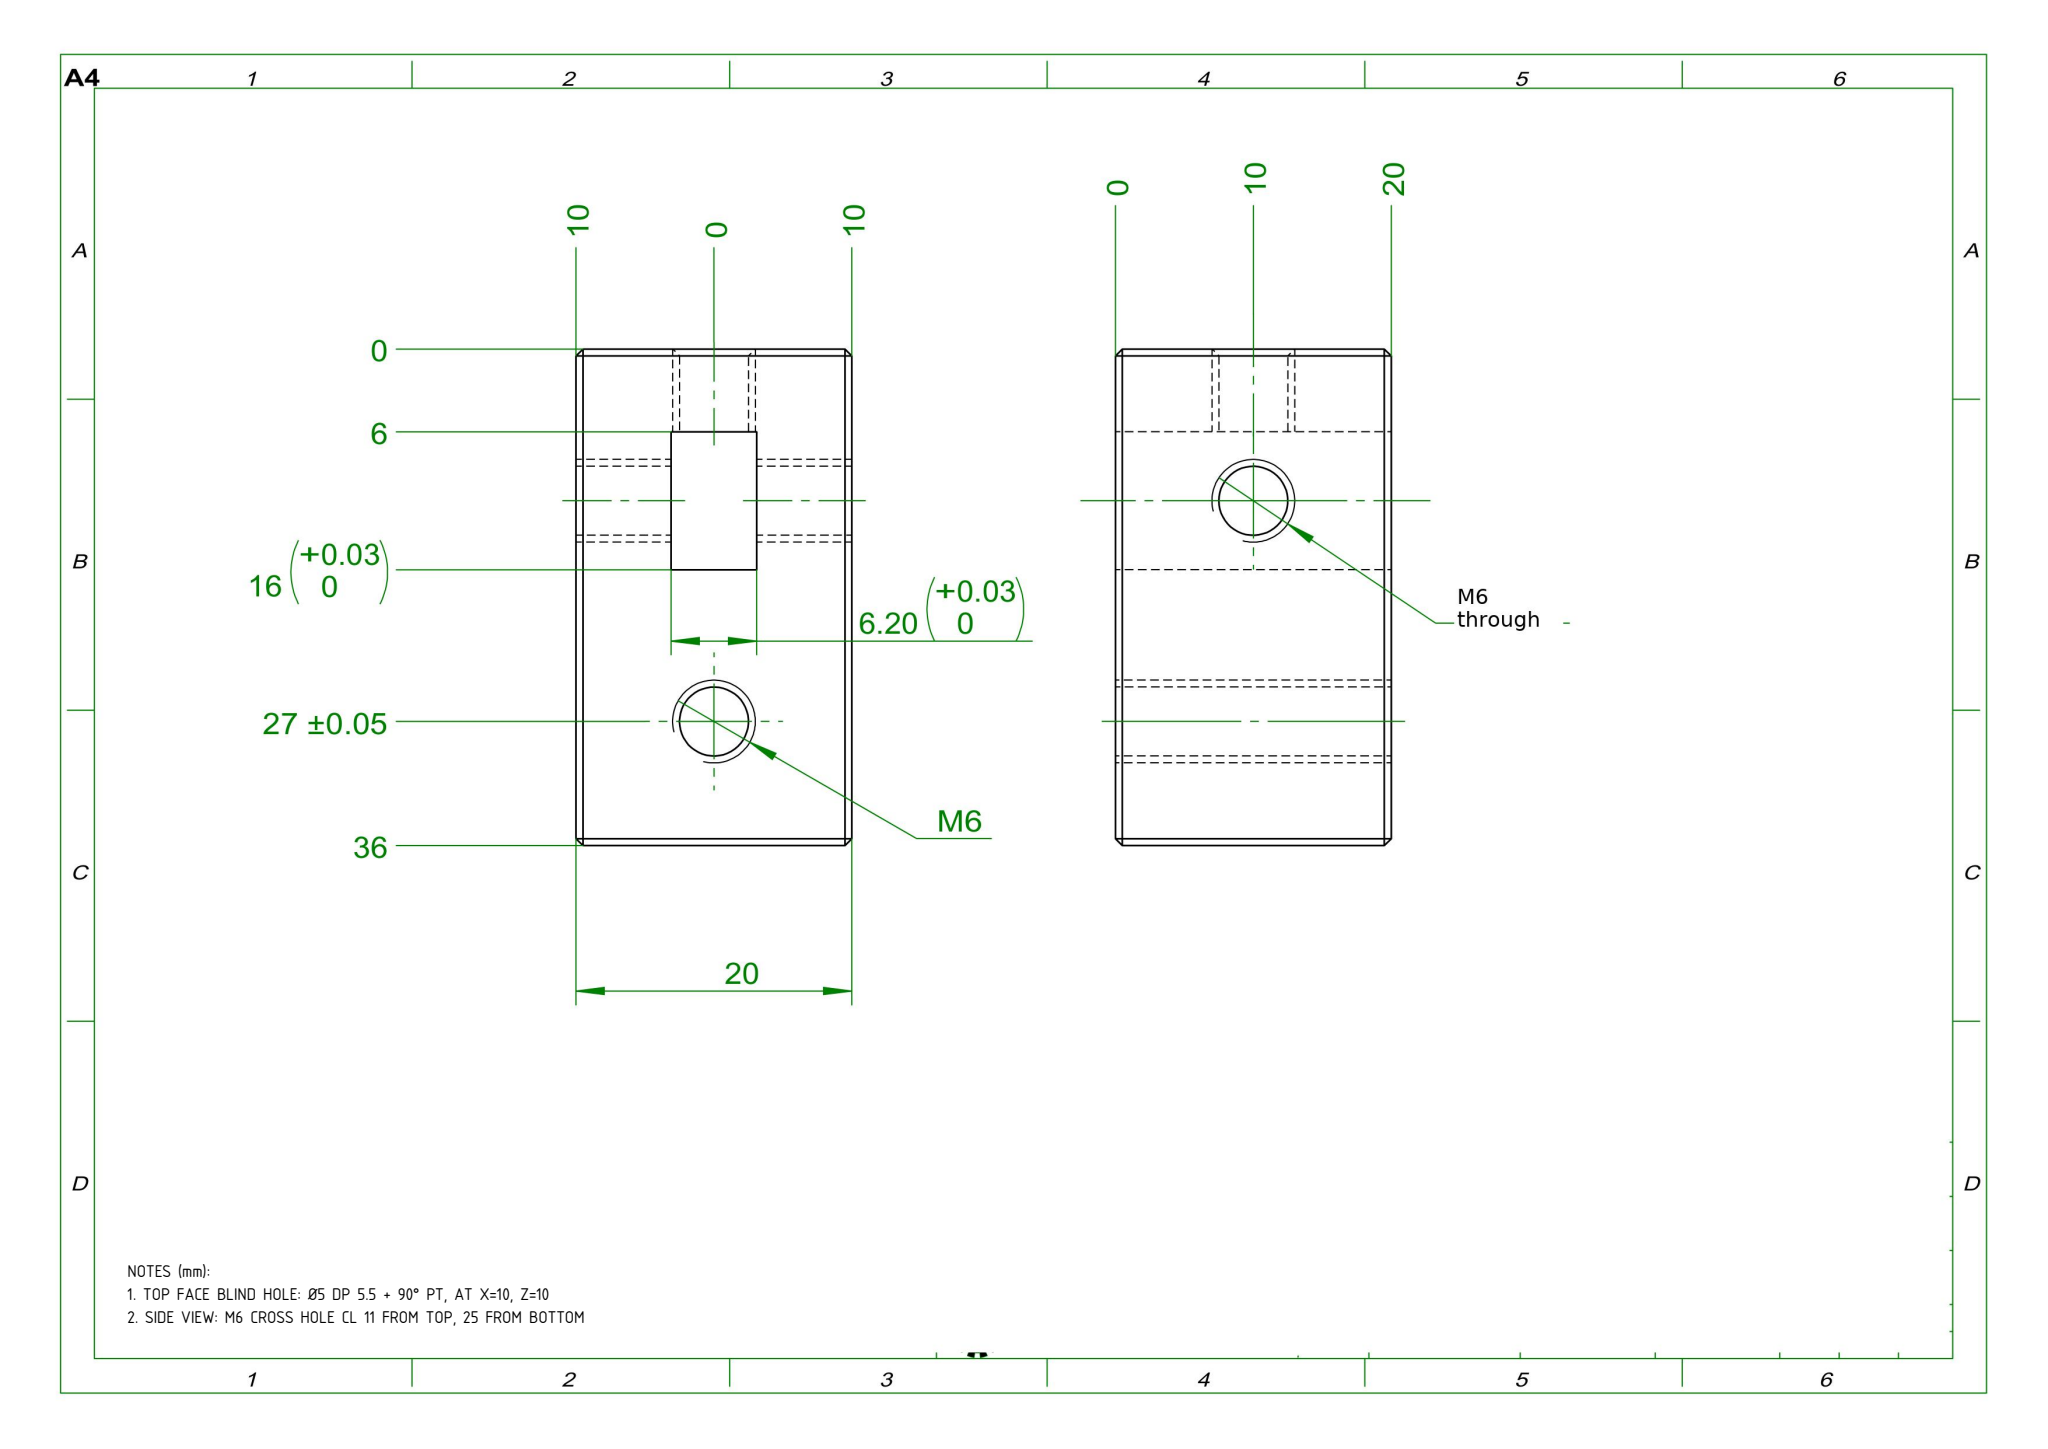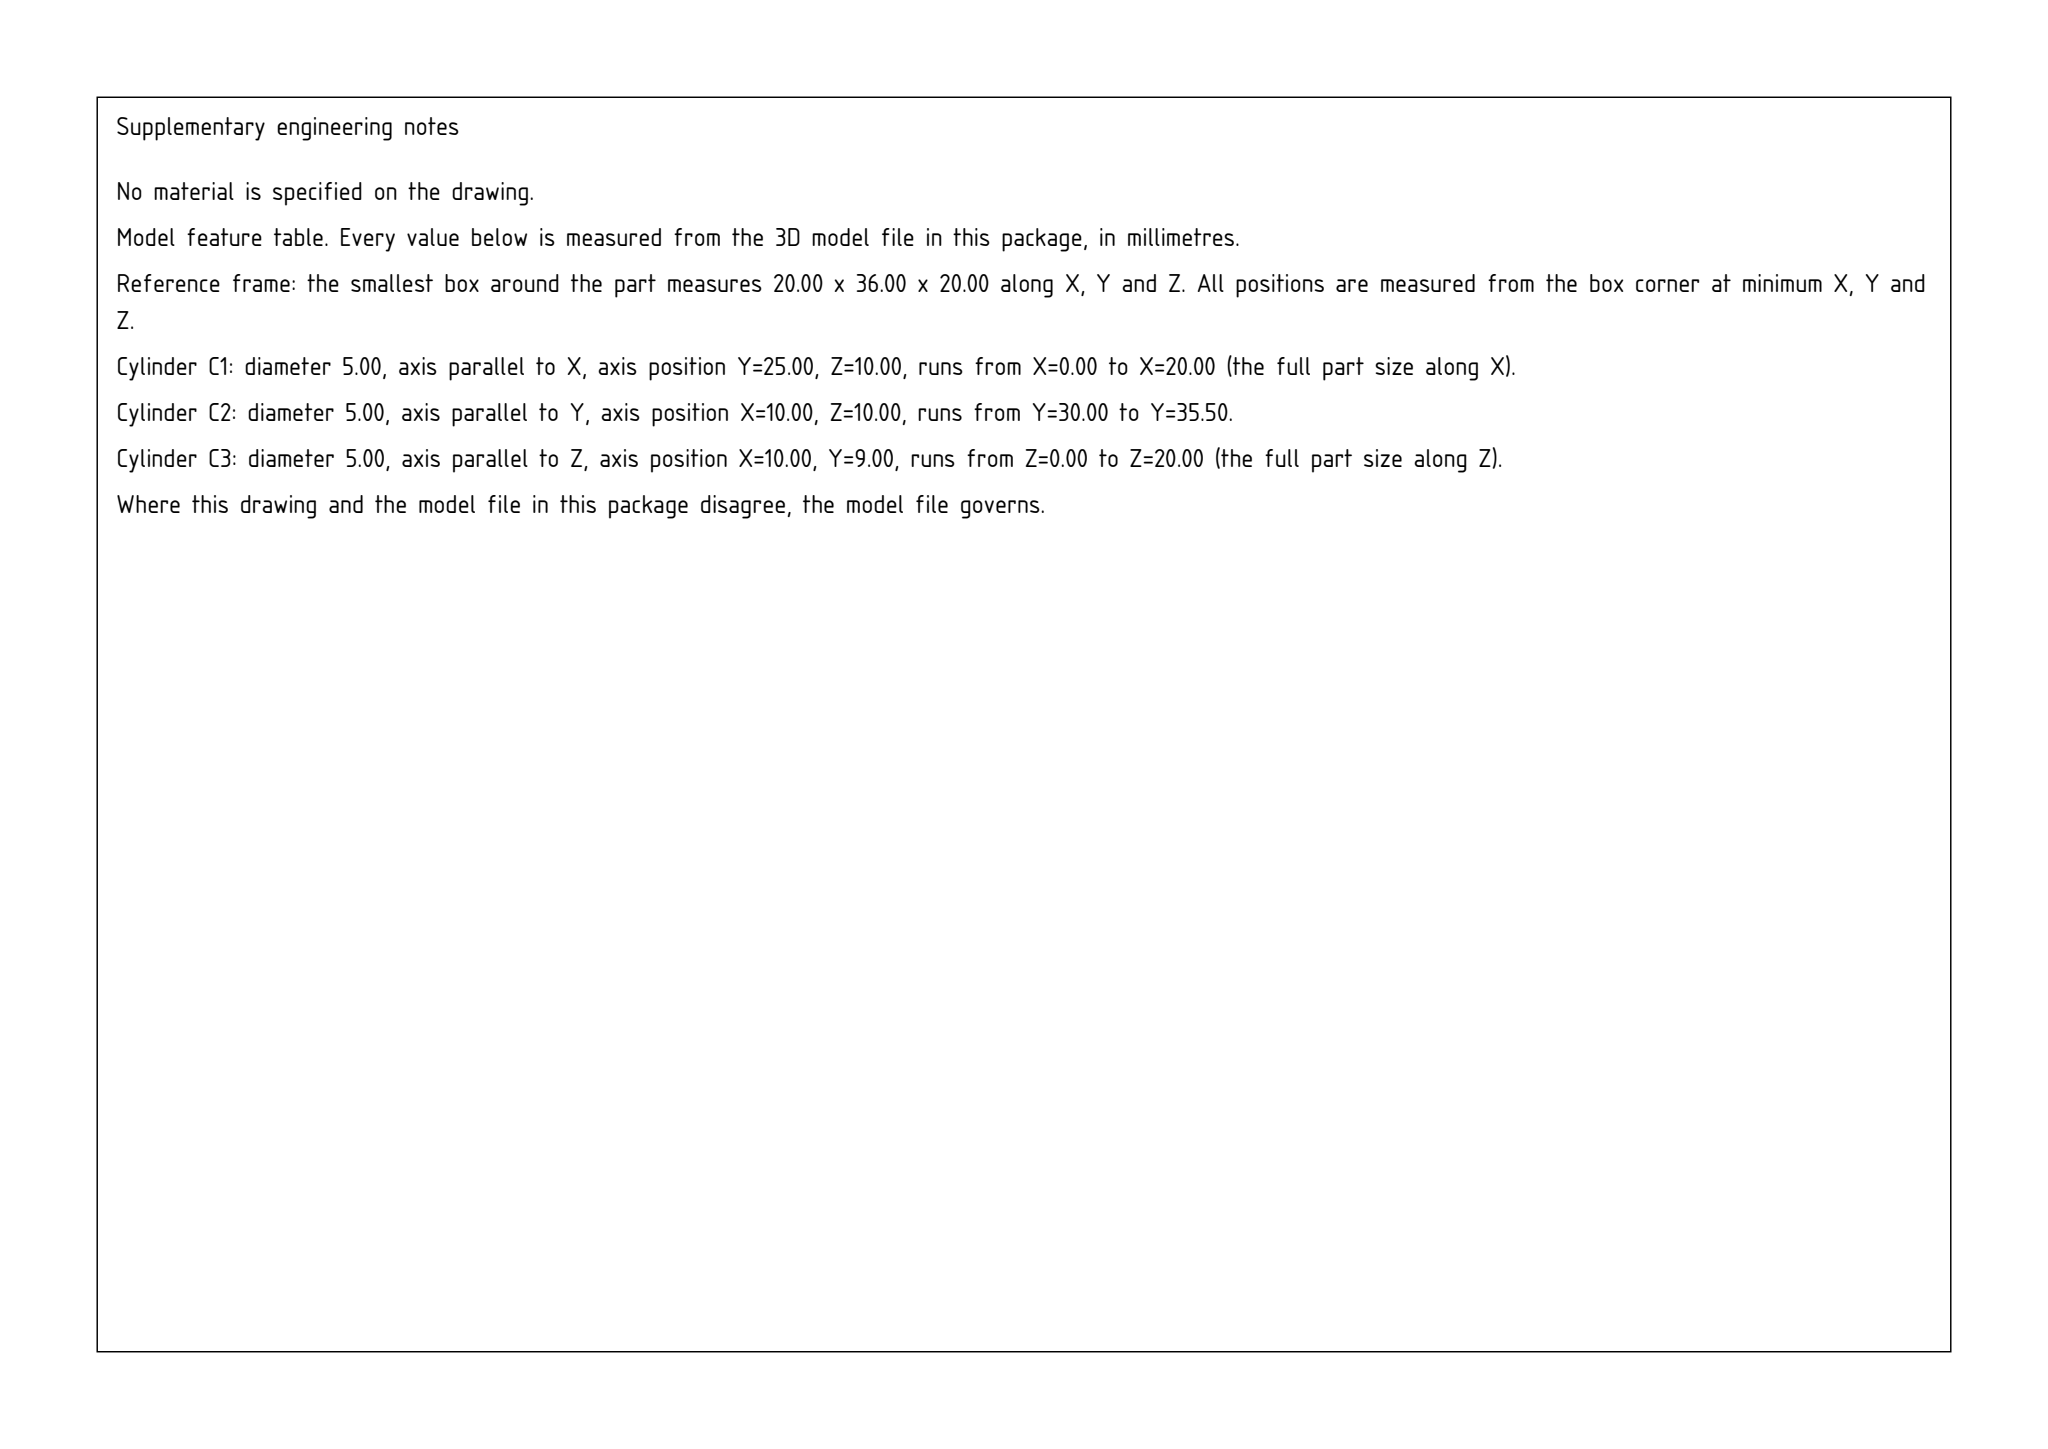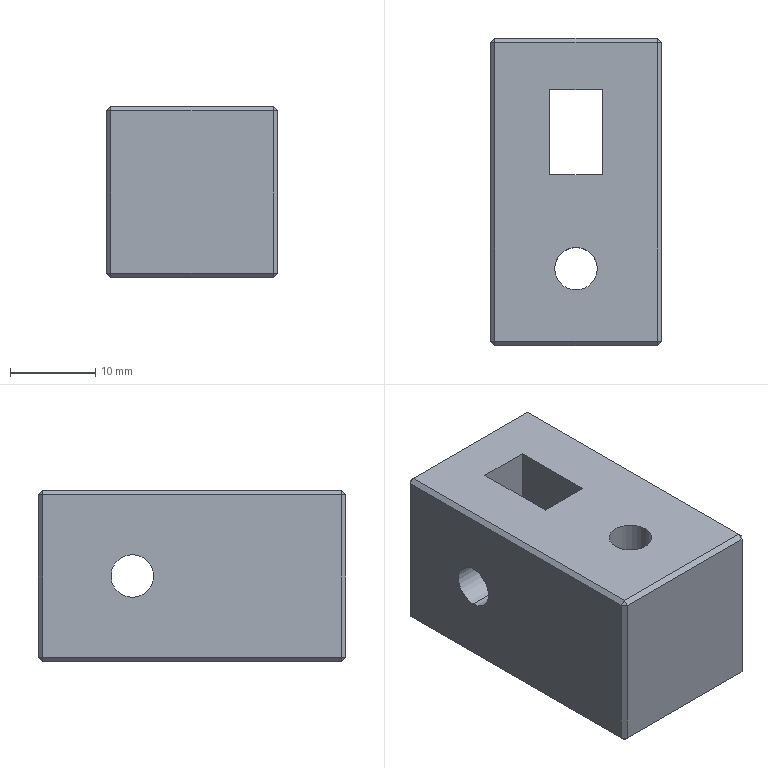Part | SolidWorks | mm | 1 solid | 40 faces | box 20 x 36 x 20 mm | volume 12339 mm3 | plane 30 | cylinder 8 | cone 2 | commonest cylinder face diameters 5 x8
Drawing notes:
TOP FACE BLIND HOLE: Ø5 DP 5.5 + 90° PT, AT X=10, Z=10 | from the solid: cylinders[5.0,'y',[10.0,null,10.0],5.5] + cone 90° ref dia 5, enters y=36 face
SIDE VIEW: M6 CROSS HOLE CL 11 FROM TOP, 25 FROM BOTTOM | from the solid: cylinders[5.0,'x',[null,25.0,10.0],6.9] -> y=25 from min = 11 from top face (y=36)
build123d program:
from build123d import *

# Parameters (mm, degrees)
SKETCH1_W             = 20
SKETCH1_H             = 36
SKETCH1_W_2           = 6.2
SKETCH1_H_2           = 10
BOSS_EXTRUDE1_DEPTH   = 20
M6_TAPPED_HOLE1_D     = 5
M6_TAPPED_HOLE1_DEPTH = 11
M6_TAPPED_HOLE1_TIP   = 1.502
CHAMFER1_SIZE         = 0.5
M6_TAPPED_HOLE2_D     = 5
M6_TAPPED_HOLE3_D     = 5


with BuildPart() as part:
    # Sketch1 → Boss-Extrude1 (new body)
    with BuildSketch(Plane.XY):
        Rectangle(SKETCH1_W, SKETCH1_H)
        with Locations((0, 7)):
            Rectangle(SKETCH1_W_2, SKETCH1_H_2, mode=Mode.SUBTRACT)
    extrude(amount=BOSS_EXTRUDE1_DEPTH)

    # M6 Tapped Hole1
    with Locations(Plane(origin=(0, 18, 0), x_dir=(1, 0, 0), z_dir=(0, 1, 0))):
        with Locations((0, -10)):
            Hole(M6_TAPPED_HOLE1_D / 2, depth=M6_TAPPED_HOLE1_DEPTH)
            with Locations((0, 0, -(M6_TAPPED_HOLE1_DEPTH + M6_TAPPED_HOLE1_TIP / 2))):  # 118° drill point
                Cone(0, M6_TAPPED_HOLE1_D / 2, M6_TAPPED_HOLE1_TIP, mode=Mode.SUBTRACT)

    # Chamfer1
    chamfer1_edges = [part.edges().sort_by_distance(p)[0] for p in [
        (-10, 0, 20),
        (0, -18, 20),
        (2.5, 18, 10),
        (10, 0, 20),
        (0, -18, 0),
        (-10, 0, 0),
        (0, 18, 0),
        (10, 0, 0),
        (0, 18, 20),
        (10, -18, 10),
        (-10, -18, 10),
        (-10, 18, 10),
        (10, 18, 10),
    ]]
    chamfer(chamfer1_edges, length=CHAMFER1_SIZE)

    # M6 Tapped Hole2 (through all)
    with Locations(Plane(origin=(0, 0, 0), x_dir=(-1, 0, 0), z_dir=(0, 0, -1))):
        with Locations((0, -9)):
            Hole(M6_TAPPED_HOLE2_D / 2)

    # M6 Tapped Hole3 (through all)
    with Locations(Plane(origin=(10, 0, 0), x_dir=(0, 0, -1), z_dir=(1, 0, 0))):
        with Locations((-10, 7)):
            Hole(M6_TAPPED_HOLE3_D / 2)


solid = part.part